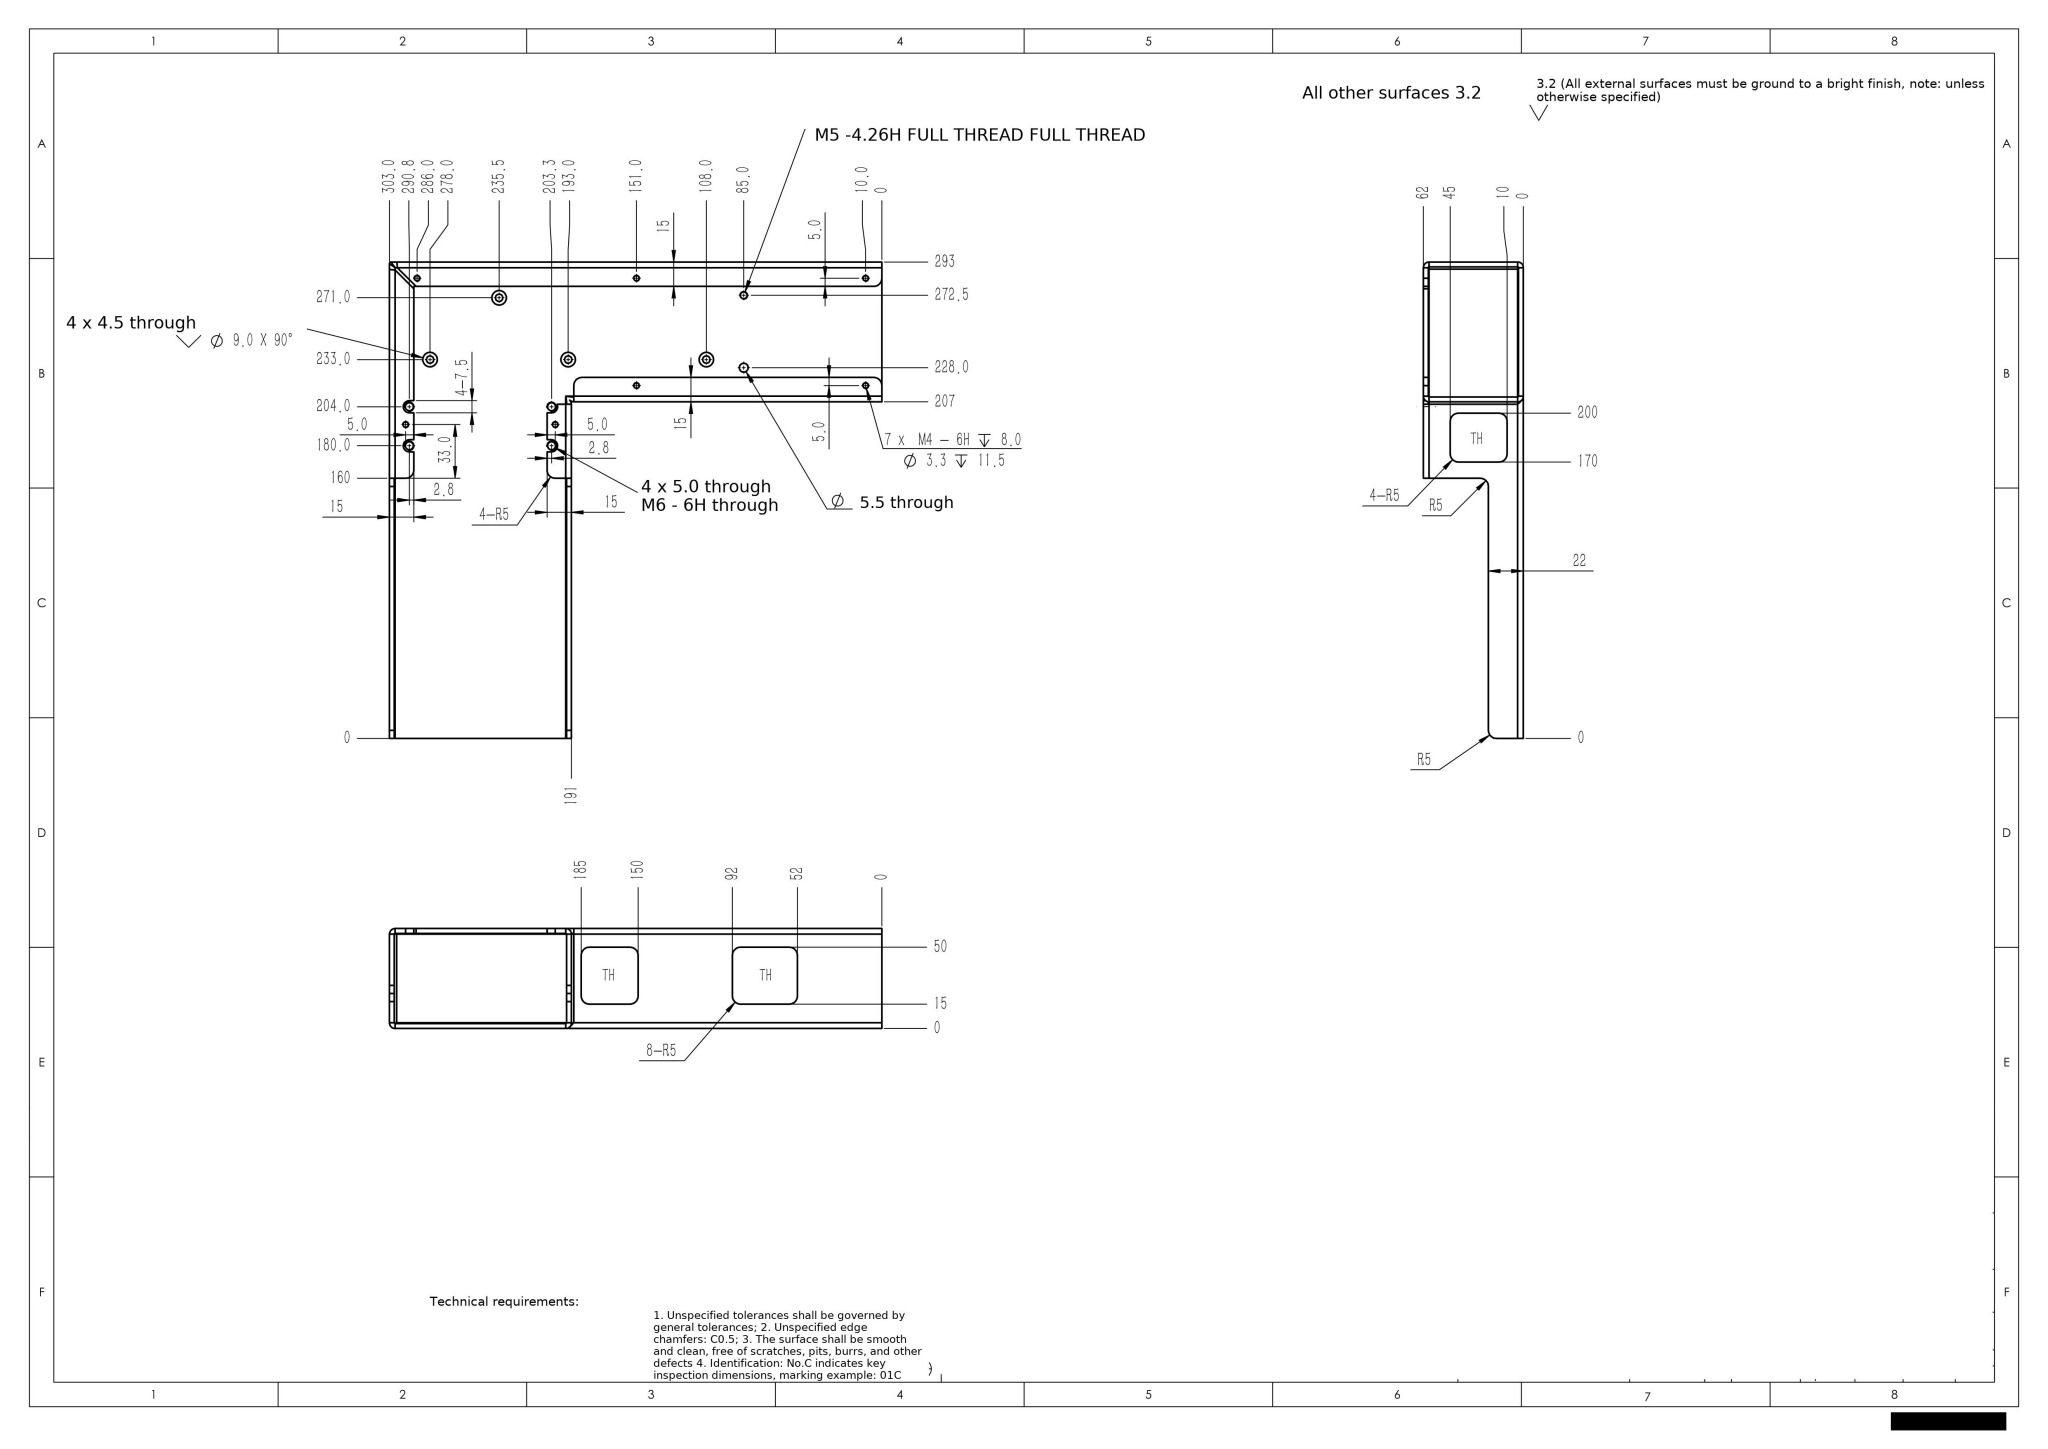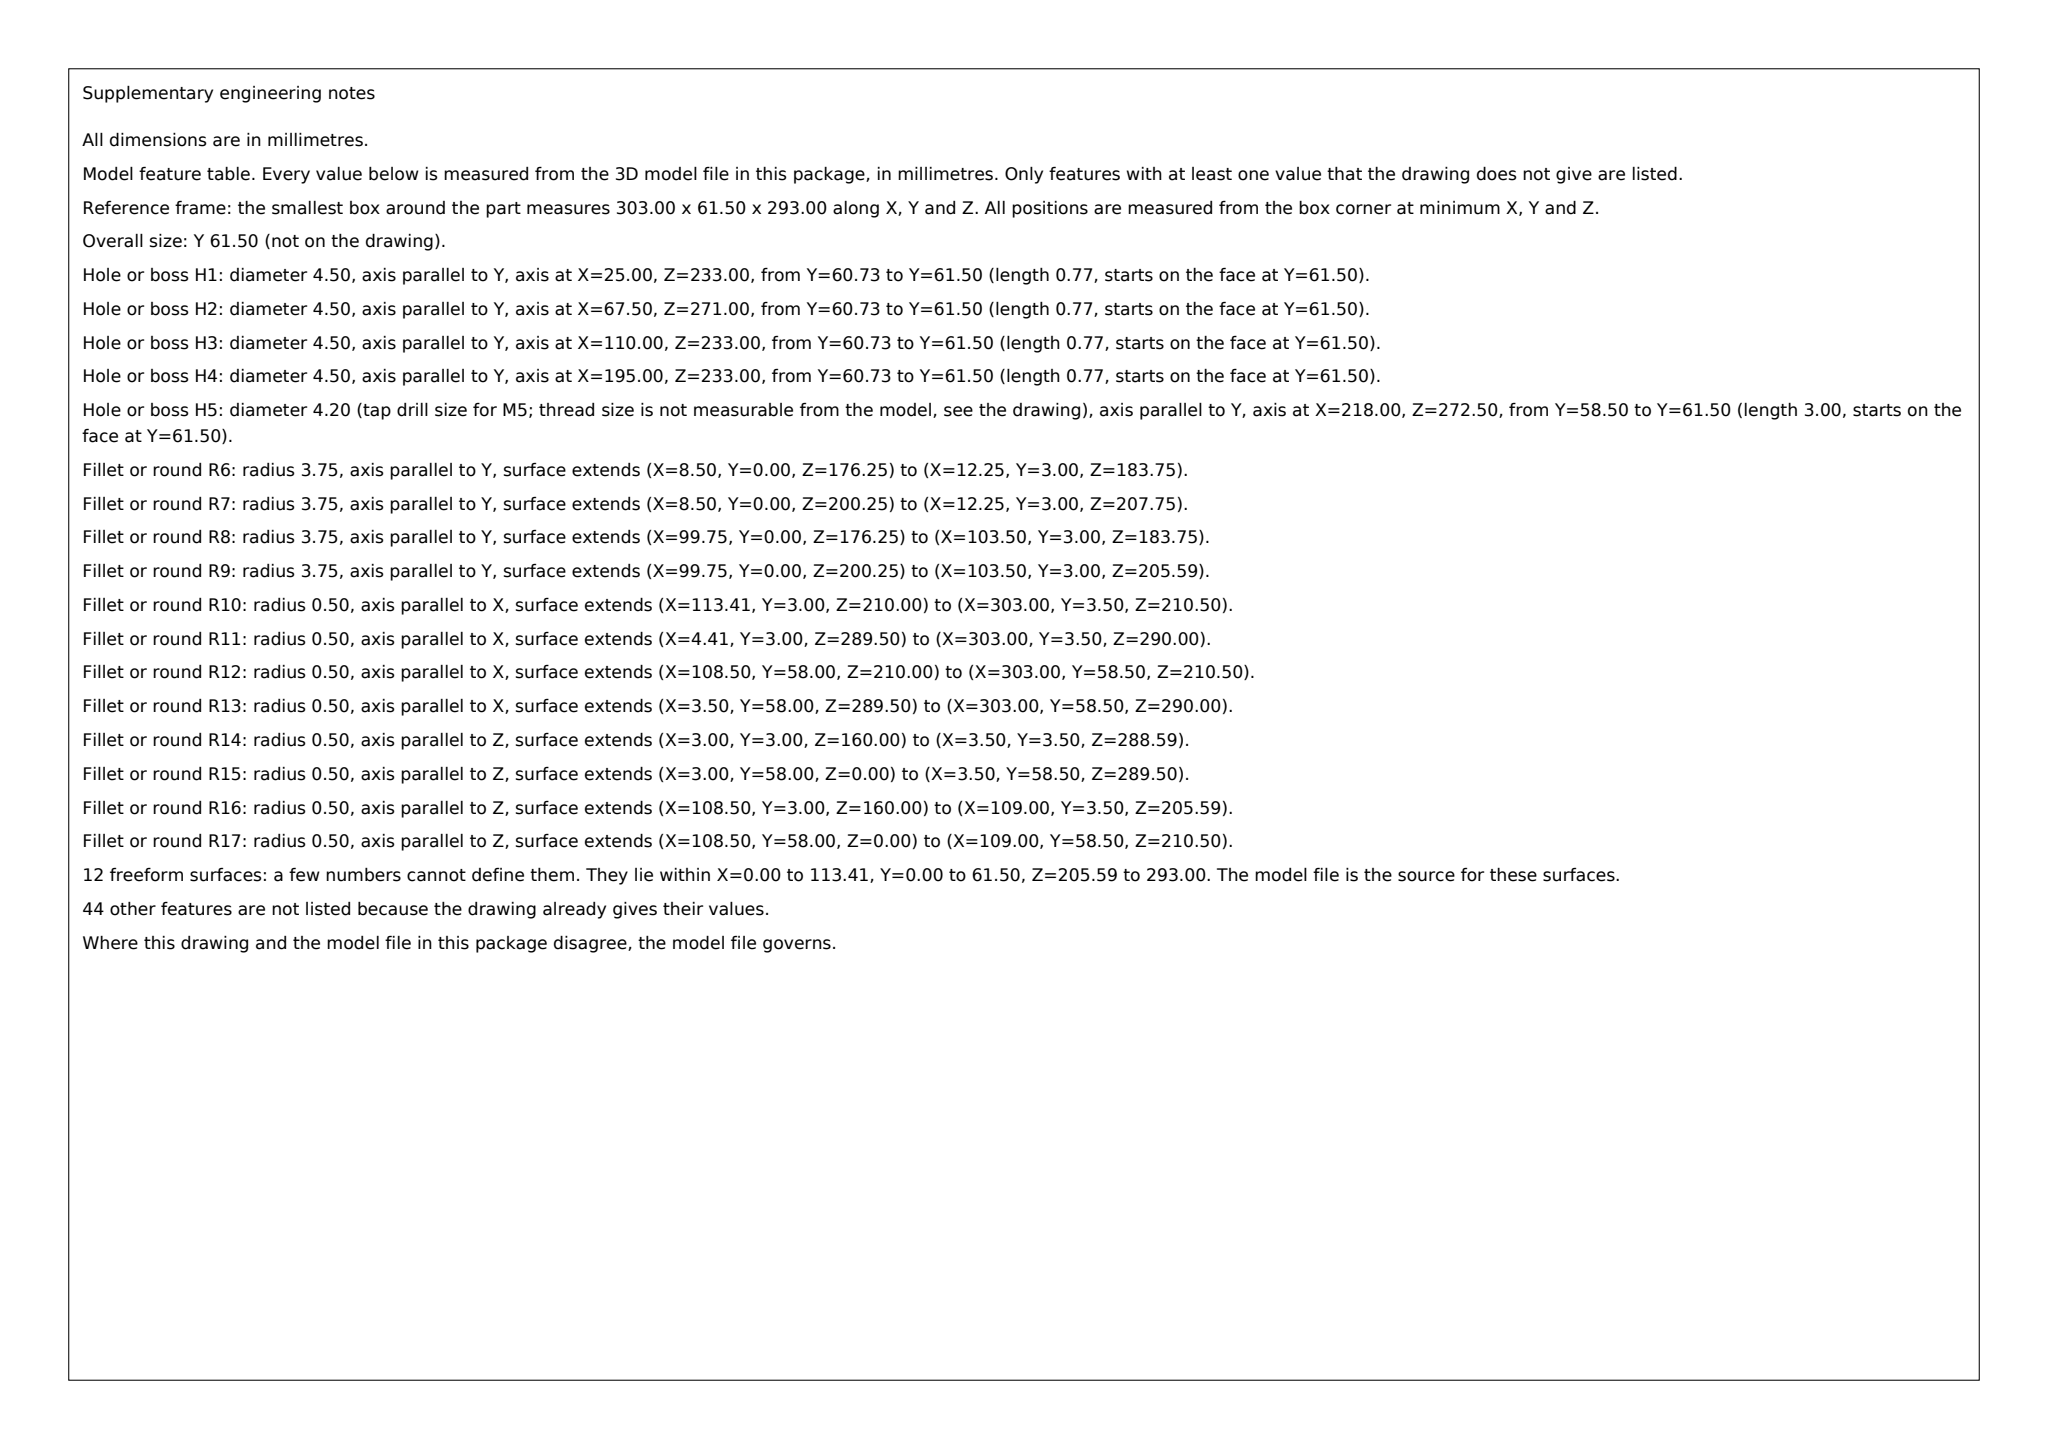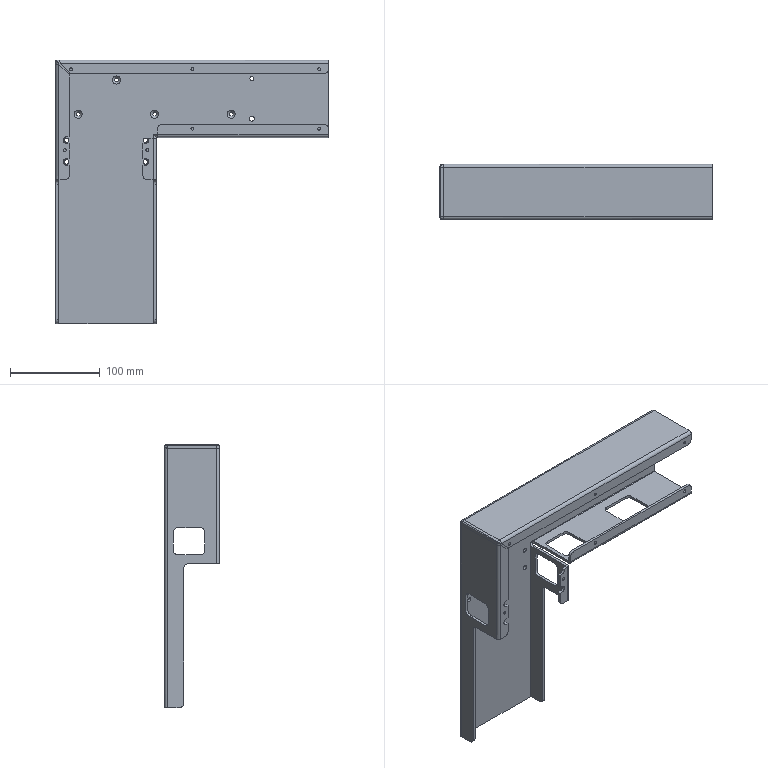Part | SolidWorks | mm | 1 solid | 186 faces | box 303 x 61.5 x 293 mm | volume 286575 mm3 | plane 84 | cylinder 82 | spline 12 | cone 8 | commonest cylinder face diameters 10 x25 3.3 x14 4.5 x8 5 x8 7 x8 1 x8 7.5 x6 4.2 x2